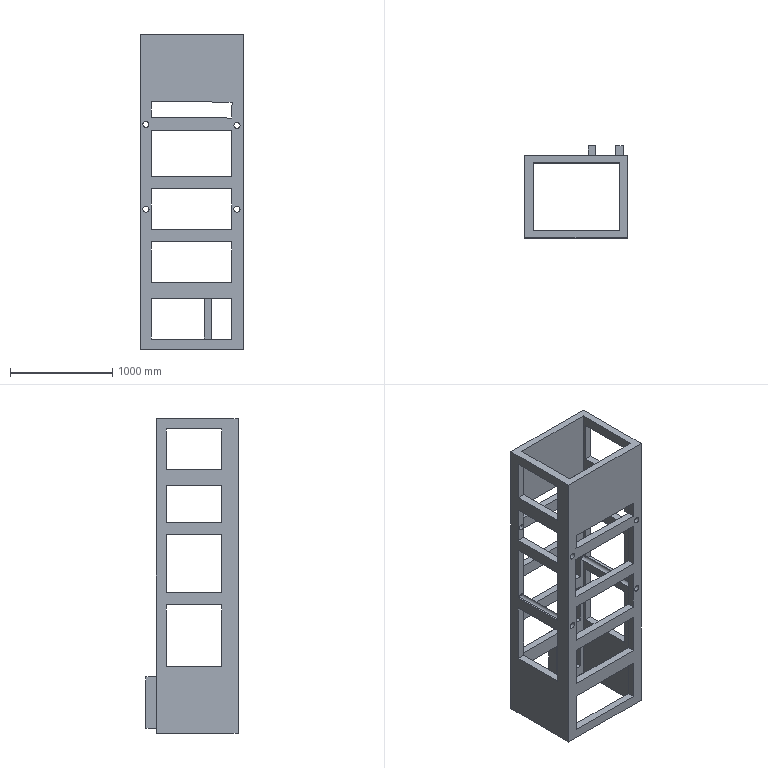Component | NX | BASE | 1 solid | 101 faces | volume 381212239 mm3 | plane 95 | cylinder 6 | commonest cylinder face diameters 60 x6